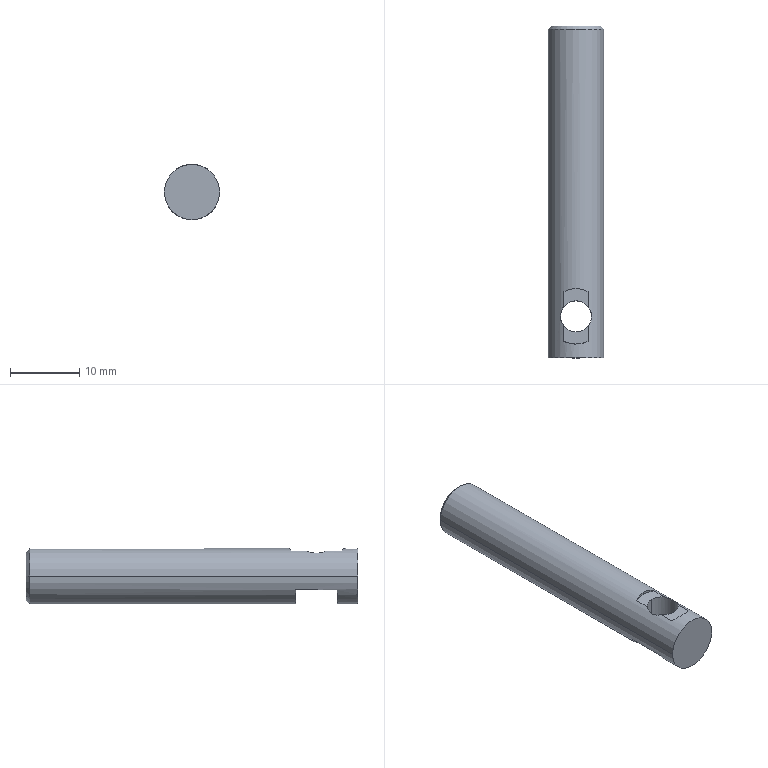Component | SolidWorks | 002MaterialPickingModuleA-1_004SidePlugModule-1_J-014-3 | 1 solid | 20 faces | box 8 x 48 x 8 mm | volume 2217 mm3 | cylinder 9 | plane 7 | cone 4 | commonest cylinder face diameters 8 x5 4.5 x2 2.5 x2 | material 45
build123d program:
from build123d import *

# Parameters (mm, degrees)
SKETCH1_R             = 4
BOSS_EXTRUDE1_DEPTH   = 48
M3_TAPPED_HOLE1_D     = 2.5
M3_TAPPED_HOLE1_DEPTH = 7.5
M3_TAPPED_HOLE1_TIP   = 0.7511
CHAMFER1_SIZE         = 0.5
SKETCH6_W             = 15
SKETCH6_H             = 6
CUT_EXTRUDE1_DEPTH    = 2


with BuildPart() as part:
    # Sketch1 → Boss-Extrude1 (new body)
    with BuildSketch(Plane.XY):
        Circle(SKETCH1_R)
    extrude(amount=BOSS_EXTRUDE1_DEPTH)

    # M3 Tapped Hole1
    with Locations(Plane(origin=(0, 0, 0), x_dir=(-1, 0, 0), z_dir=(0, 0, -1))):
        with Locations((0, 0)):
            Hole(M3_TAPPED_HOLE1_D / 2, depth=M3_TAPPED_HOLE1_DEPTH)
            with Locations((0, 0, -(M3_TAPPED_HOLE1_DEPTH + M3_TAPPED_HOLE1_TIP / 2))):  # 118° drill point
                Cone(0, M3_TAPPED_HOLE1_D / 2, M3_TAPPED_HOLE1_TIP, mode=Mode.SUBTRACT)

    # Chamfer1
    chamfer1_edges = [part.edges().sort_by_distance(p)[0] for p in [
        (-4, 0, 0),
    ]]
    chamfer(chamfer1_edges, length=CHAMFER1_SIZE)

    # Sketch6 → Cut-Extrude1 (cut)
    with BuildSketch(Plane(origin=(0, 4, 0), x_dir=(1, 0, 0), z_dir=(0, 1, 0))):
        with Locations((0, -42)):
            Rectangle(SKETCH6_W, SKETCH6_H)
    extrude(amount=-CUT_EXTRUDE1_DEPTH, mode=Mode.SUBTRACT)

    # Sketch8 → M4 Hex Socket Head Cap Screw CBORE1 (revolve, cut)
    with BuildSketch(Plane(origin=(0, -8, 42), x_dir=(0, 0, -1), z_dir=(1, 0, 0))):
        Polygon((0, 0), (0, 12), (2.25, 12), (2.25, 4.4), (4, 4.4), (4, 0.025), (4.025, 0), align=None)
    revolve(axis=Axis((0, -14.35, 42), (0, 1, 0)), mode=Mode.SUBTRACT)


solid = part.part

# Placed as in the assembly
solid = solid.moved(Location((95.325, 338.019, 464.731), (90, 0, -180)))
STEP:
#1=CARTESIAN_POINT('',(3.753,11.743,18.218));
#2=VERTEX_POINT('',#1);
#3=CARTESIAN_POINT('',(3.753,11.566,18.218));
#4=VERTEX_POINT('',#3);
#5=CARTESIAN_POINT('',(3.753,11.654,18.218));
#6=DIRECTION('',(0.,-0.,-1.));
#7=DIRECTION('',(0.,-1.,0.));
#8=AXIS2_PLACEMENT_3D('',#5,#6,#7);
#9=CIRCLE('',#8,0.08858);
#10=EDGE_CURVE('',#2,#4,#9,.T.);
#11=ORIENTED_EDGE('',*,*,#10,.T.);
#12=CARTESIAN_POINT('',(3.753,11.566,18.438));
#13=VERTEX_POINT('',#12);
#14=CARTESIAN_POINT('',(3.753,11.566,18.611));
#15=DIRECTION('',(-0.,0.,1.));
#16=VECTOR('',#15,39.37);
#17=LINE('',#14,#16);
#18=EDGE_CURVE('',#4,#13,#17,.T.);
#19=ORIENTED_EDGE('',*,*,#18,.T.);
#20=CARTESIAN_POINT('',(3.822,11.598,18.438));
#21=VERTEX_POINT('',#20);
#22=CARTESIAN_POINT('',(3.753,11.654,18.438));
#23=DIRECTION('',(-0.,0.,1.));
#24=DIRECTION('',(0.,1.,0.));
#25=AXIS2_PLACEMENT_3D('',#22,#23,#24);
#26=CIRCLE('',#25,0.08858);
#27=EDGE_CURVE('',#13,#21,#26,.T.);
#28=ORIENTED_EDGE('',*,*,#27,.T.);
#29=CARTESIAN_POINT('',(3.822,11.71,18.438));
#30=VERTEX_POINT('',#29);
#31=CARTESIAN_POINT('',(3.822,11.71,18.438));
#32=CARTESIAN_POINT('',(3.828,11.703,18.435));
#33=CARTESIAN_POINT('',(3.833,11.694,18.432));
#34=CARTESIAN_POINT('',(3.838,11.68,18.429));
#35=CARTESIAN_POINT('',(3.839,11.675,18.428));
#36=CARTESIAN_POINT('',(3.841,11.665,18.427));
#37=CARTESIAN_POINT('',(3.842,11.66,18.427));
#38=CARTESIAN_POINT('',(3.842,11.649,18.427));
#39=CARTESIAN_POINT('',(3.841,11.644,18.427));
#40=CARTESIAN_POINT('',(3.839,11.634,18.428));
#41=CARTESIAN_POINT('',(3.838,11.629,18.429));
#42=CARTESIAN_POINT('',(3.833,11.615,18.432));
#43=CARTESIAN_POINT('',(3.828,11.606,18.435));
#44=CARTESIAN_POINT('',(3.822,11.598,18.438));
#45=B_SPLINE_CURVE_WITH_KNOTS('',3,(#31,#32,#33,#34,#35,#36,#37,#38,#39,#40,#41,#42,#43,#44),.UNSPECIFIED.,.F.,.F.,(4,2,2,2,2,2,4),(0.,0.0007826,0.001174,0.001565,0.001957,0.002348,0.00313),.UNSPECIFIED.);
#46=EDGE_CURVE('',#30,#21,#45,.T.);
#47=ORIENTED_EDGE('',*,*,#46,.F.);
#48=CARTESIAN_POINT('',(3.753,11.743,18.438));
#49=VERTEX_POINT('',#48);
#50=CARTESIAN_POINT('',(3.753,11.654,18.438));
#51=DIRECTION('',(-0.,0.,1.));
#52=DIRECTION('',(0.,1.,0.));
#53=AXIS2_PLACEMENT_3D('',#50,#51,#52);
#54=CIRCLE('',#53,0.08858);
#55=EDGE_CURVE('',#30,#49,#54,.T.);
#56=ORIENTED_EDGE('',*,*,#55,.T.);
#57=CARTESIAN_POINT('',(3.753,11.743,18.611));
#58=DIRECTION('',(-0.,0.,1.));
#59=VECTOR('',#58,39.37);
#60=LINE('',#57,#59);
#61=EDGE_CURVE('',#2,#49,#60,.T.);
#62=ORIENTED_EDGE('',*,*,#61,.F.);
#63=EDGE_LOOP('',(#11,#19,#28,#47,#56,#62));
#64=FACE_OUTER_BOUND('',#63,.T.);
#65=CARTESIAN_POINT('',(3.753,11.654,18.611));
#66=DIRECTION('',(-0.,0.,1.));
#67=DIRECTION('',(0.,1.,0.));
#68=AXIS2_PLACEMENT_3D('',#65,#66,#67);
#69=CYLINDRICAL_SURFACE('',#68,0.08858);
#70=ADVANCED_FACE('',(#64),#69,.F.);
#71=CARTESIAN_POINT('',(3.753,11.812,18.438));
#72=VERTEX_POINT('',#71);
#73=CARTESIAN_POINT('',(3.684,11.796,18.438));
#74=VERTEX_POINT('',#73);
#75=CARTESIAN_POINT('',(3.753,11.654,18.438));
#76=DIRECTION('',(-0.,0.,1.));
#77=DIRECTION('',(0.,1.,0.));
#78=AXIS2_PLACEMENT_3D('',#75,#76,#77);
#79=CIRCLE('',#78,0.1575);
#80=EDGE_CURVE('',#72,#74,#79,.T.);
#81=ORIENTED_EDGE('',*,*,#80,.F.);
#82=CARTESIAN_POINT('',(3.753,11.812,18.454));
#83=VERTEX_POINT('',#82);
#84=CARTESIAN_POINT('',(3.753,11.812,18.611));
#85=DIRECTION('',(-0.,0.,1.));
#86=VECTOR('',#85,39.37);
#87=LINE('',#84,#86);
#88=EDGE_CURVE('',#72,#83,#87,.T.);
#89=ORIENTED_EDGE('',*,*,#88,.T.);
#90=CARTESIAN_POINT('',(3.684,11.796,18.438));
#91=CARTESIAN_POINT('',(3.706,11.806,18.449));
#92=CARTESIAN_POINT('',(3.729,11.812,18.454));
#93=CARTESIAN_POINT('',(3.753,11.812,18.454));
#94=(BOUNDED_CURVE()B_SPLINE_CURVE(3,(#90,#91,#92,#93),.UNSPECIFIED.,.F.,.F.)B_SPLINE_CURVE_WITH_KNOTS((4,4),(5.832,6.283),.UNSPECIFIED.)CURVE()GEOMETRIC_REPRESENTATION_ITEM()RATIONAL_B_SPLINE_CURVE((1.,0.9831,0.9831,1.))REPRESENTATION_ITEM(''));
#95=EDGE_CURVE('',#74,#83,#94,.T.);
#96=ORIENTED_EDGE('',*,*,#95,.F.);
#97=EDGE_LOOP('',(#81,#89,#96));
#98=FACE_OUTER_BOUND('',#97,.T.);
#99=CARTESIAN_POINT('',(3.753,11.654,18.611));
#100=DIRECTION('',(-0.,0.,1.));
#101=DIRECTION('',(0.,1.,0.));
#102=AXIS2_PLACEMENT_3D('',#99,#100,#101);
#103=CYLINDRICAL_SURFACE('',#102,0.1575);
#104=ADVANCED_FACE('',(#98),#103,.F.);
#105=CARTESIAN_POINT('',(3.891,13.308,18.296));
#106=VERTEX_POINT('',#105);
#107=CARTESIAN_POINT('',(3.615,13.308,18.296));
#108=VERTEX_POINT('',#107);
#109=CARTESIAN_POINT('',(3.753,13.308,18.296));
#110=DIRECTION('',(-0.,1.,-0.));
#111=DIRECTION('',(-1.,0.,0.));
#112=AXIS2_PLACEMENT_3D('',#109,#110,#111);
#113=CIRCLE('',#112,0.1378);
#114=EDGE_CURVE('',#106,#108,#113,.T.);
#115=ORIENTED_EDGE('',*,*,#114,.F.);
#116=CARTESIAN_POINT('',(3.91,13.288,18.296));
#117=VERTEX_POINT('',#116);
#118=CARTESIAN_POINT('',(3.91,13.288,18.296));
#119=DIRECTION('',(0.7071,-0.7071,-0.));
#120=VECTOR('',#119,39.37);
#121=LINE('',#118,#120);
#122=EDGE_CURVE('',#106,#117,#121,.T.);
#123=ORIENTED_EDGE('',*,*,#122,.T.);
#124=CARTESIAN_POINT('',(3.595,13.288,18.296));
#125=VERTEX_POINT('',#124);
#126=CARTESIAN_POINT('',(3.753,13.288,18.296));
#127=DIRECTION('',(0.,-1.,0.));
#128=DIRECTION('',(-1.,0.,0.));
#129=AXIS2_PLACEMENT_3D('',#126,#127,#128);
#130=CIRCLE('',#129,0.1575);
#131=EDGE_CURVE('',#125,#117,#130,.T.);
#132=ORIENTED_EDGE('',*,*,#131,.F.);
#133=CARTESIAN_POINT('',(3.595,13.288,18.296));
#134=DIRECTION('',(-0.7071,-0.7071,0.));
#135=VECTOR('',#134,39.37);
#136=LINE('',#133,#135);
#137=EDGE_CURVE('',#108,#125,#136,.T.);
#138=ORIENTED_EDGE('',*,*,#137,.F.);
#139=EDGE_LOOP('',(#115,#123,#132,#138));
#140=FACE_OUTER_BOUND('',#139,.T.);
#141=CARTESIAN_POINT('',(3.753,13.288,18.296));
#142=DIRECTION('',(0.,-1.,0.));
#143=DIRECTION('',(-1.,0.,0.));
#144=AXIS2_PLACEMENT_3D('',#141,#142,#143);
#145=CONICAL_SURFACE('',#144,0.1575,0.7854);
#146=ADVANCED_FACE('',(#140),#145,.T.);
#147=CARTESIAN_POINT('',(3.704,13.013,18.296));
#148=VERTEX_POINT('',#147);
#149=CARTESIAN_POINT('',(3.802,13.013,18.296));
#150=VERTEX_POINT('',#149);
#151=CARTESIAN_POINT('',(3.753,13.013,18.296));
#152=DIRECTION('',(-0.,1.,-0.));
#153=DIRECTION('',(1.,0.,0.));
#154=AXIS2_PLACEMENT_3D('',#151,#152,#153);
#155=CIRCLE('',#154,0.04921);
#156=EDGE_CURVE('',#148,#150,#155,.T.);
#157=ORIENTED_EDGE('',*,*,#156,.F.);
#158=CARTESIAN_POINT('',(3.704,13.308,18.296));
#159=VERTEX_POINT('',#158);
#160=CARTESIAN_POINT('',(3.704,13.308,18.296));
#161=DIRECTION('',(-0.,1.,-0.));
#162=VECTOR('',#161,39.37);
#163=LINE('',#160,#162);
#164=EDGE_CURVE('',#148,#159,#163,.T.);
#165=ORIENTED_EDGE('',*,*,#164,.T.);
#166=CARTESIAN_POINT('',(3.802,13.308,18.296));
#167=VERTEX_POINT('',#166);
#168=CARTESIAN_POINT('',(3.753,13.308,18.296));
#169=DIRECTION('',(-0.,1.,-0.));
#170=DIRECTION('',(1.,0.,0.));
#171=AXIS2_PLACEMENT_3D('',#168,#169,#170);
#172=CIRCLE('',#171,0.04921);
#173=EDGE_CURVE('',#159,#167,#172,.T.);
#174=ORIENTED_EDGE('',*,*,#173,.T.);
#175=CARTESIAN_POINT('',(3.802,13.308,18.296));
#176=DIRECTION('',(-0.,1.,-0.));
#177=VECTOR('',#176,39.37);
#178=LINE('',#175,#177);
#179=EDGE_CURVE('',#150,#167,#178,.T.);
#180=ORIENTED_EDGE('',*,*,#179,.F.);
#181=EDGE_LOOP('',(#157,#165,#174,#180));
#182=FACE_OUTER_BOUND('',#181,.T.);
#183=CARTESIAN_POINT('',(3.753,13.308,18.296));
#184=DIRECTION('',(-0.,1.,-0.));
#185=DIRECTION('',(1.,0.,0.));
#186=AXIS2_PLACEMENT_3D('',#183,#184,#185);
#187=CYLINDRICAL_SURFACE('',#186,0.04921);
#188=ADVANCED_FACE('',(#182),#187,.F.);
#189=CARTESIAN_POINT('',(3.753,12.983,18.296));
#190=VERTEX_POINT('',#189);
#191=CARTESIAN_POINT('',(3.802,13.013,18.296));
#192=DIRECTION('',(0.8572,0.515,-0.));
#193=VECTOR('',#192,39.37);
#194=LINE('',#191,#193);
#195=EDGE_CURVE('',#190,#150,#194,.T.);
#196=ORIENTED_EDGE('',*,*,#195,.F.);
#197=CARTESIAN_POINT('',(3.704,13.013,18.296));
#198=DIRECTION('',(-0.8572,0.515,-0.));
#199=VECTOR('',#198,39.37);
#200=LINE('',#197,#199);
#201=EDGE_CURVE('',#190,#148,#200,.T.);
#202=ORIENTED_EDGE('',*,*,#201,.T.);
#203=ORIENTED_EDGE('',*,*,#156,.T.);
#204=EDGE_LOOP('',(#196,#202,#203));
#205=FACE_OUTER_BOUND('',#204,.T.);
#206=CARTESIAN_POINT('',(3.753,13.013,18.296));
#207=DIRECTION('',(-0.,1.,-0.));
#208=DIRECTION('',(1.,0.,0.));
#209=AXIS2_PLACEMENT_3D('',#206,#207,#208);
#210=CONICAL_SURFACE('',#209,0.04921,1.03);
#211=ADVANCED_FACE('',(#205),#210,.F.);
#212=CARTESIAN_POINT('',(3.889,11.772,18.218));
#213=VERTEX_POINT('',#212);
#214=CARTESIAN_POINT('',(3.889,11.536,18.218));
#215=VERTEX_POINT('',#214);
#216=CARTESIAN_POINT('',(3.889,11.418,18.218));
#217=DIRECTION('',(0.,-1.,0.));
#218=VECTOR('',#217,39.37);
#219=LINE('',#216,#218);
#220=EDGE_CURVE('',#213,#215,#219,.T.);
#221=ORIENTED_EDGE('',*,*,#220,.F.);
#222=CARTESIAN_POINT('',(3.617,11.772,18.218));
#223=VERTEX_POINT('',#222);
#224=CARTESIAN_POINT('',(3.753,11.772,18.296));
#225=DIRECTION('',(-0.,1.,-0.));
#226=DIRECTION('',(1.,0.,0.));
#227=AXIS2_PLACEMENT_3D('',#224,#225,#226);
#228=CIRCLE('',#227,0.1575);
#229=EDGE_CURVE('',#213,#223,#228,.T.);
#230=ORIENTED_EDGE('',*,*,#229,.T.);
#231=CARTESIAN_POINT('',(3.617,11.536,18.218));
#232=VERTEX_POINT('',#231);
#233=CARTESIAN_POINT('',(3.617,11.418,18.218));
#234=DIRECTION('',(-0.,1.,-0.));
#235=VECTOR('',#234,39.37);
#236=LINE('',#233,#235);
#237=EDGE_CURVE('',#232,#223,#236,.T.);
#238=ORIENTED_EDGE('',*,*,#237,.F.);
#239=CARTESIAN_POINT('',(3.753,11.536,18.296));
#240=DIRECTION('',(0.,-1.,0.));
#241=DIRECTION('',(-1.,0.,0.));
#242=AXIS2_PLACEMENT_3D('',#239,#240,#241);
#243=CIRCLE('',#242,0.1575);
#244=EDGE_CURVE('',#232,#215,#243,.T.);
#245=ORIENTED_EDGE('',*,*,#244,.T.);
#246=EDGE_LOOP('',(#221,#230,#238,#245));
#247=FACE_BOUND('',#246,.T.);
#248=CARTESIAN_POINT('',(3.595,11.418,18.296));
#249=VERTEX_POINT('',#248);
#250=CARTESIAN_POINT('',(3.91,11.418,18.296));
#251=VERTEX_POINT('',#250);
#252=CARTESIAN_POINT('',(3.753,11.418,18.296));
#253=DIRECTION('',(0.,-1.,0.));
#254=DIRECTION('',(-1.,0.,0.));
#255=AXIS2_PLACEMENT_3D('',#252,#253,#254);
#256=CIRCLE('',#255,0.1575);
#257=EDGE_CURVE('',#249,#251,#256,.T.);
#258=ORIENTED_EDGE('',*,*,#257,.F.);
#259=CARTESIAN_POINT('',(3.595,11.418,18.296));
#260=DIRECTION('',(-0.,1.,-0.));
#261=VECTOR('',#260,39.37);
#262=LINE('',#259,#261);
#263=EDGE_CURVE('',#249,#125,#262,.T.);
#264=ORIENTED_EDGE('',*,*,#263,.T.);
#265=ORIENTED_EDGE('',*,*,#131,.T.);
#266=CARTESIAN_POINT('',(3.91,11.418,18.296));
#267=DIRECTION('',(-0.,1.,-0.));
#268=VECTOR('',#267,39.37);
#269=LINE('',#266,#268);
#270=EDGE_CURVE('',#251,#117,#269,.T.);
#271=ORIENTED_EDGE('',*,*,#270,.F.);
#272=EDGE_LOOP('',(#258,#264,#265,#271));
#273=FACE_OUTER_BOUND('',#272,.T.);
#274=CARTESIAN_POINT('',(3.753,11.418,18.296));
#275=DIRECTION('',(-0.,1.,-0.));
#276=DIRECTION('',(1.,0.,0.));
#277=AXIS2_PLACEMENT_3D('',#274,#275,#276);
#278=CYLINDRICAL_SURFACE('',#277,0.1575);
#279=ADVANCED_FACE('',(#247,#273),#278,.T.);
#280=ORIENTED_EDGE('',*,*,#263,.F.);
#281=CARTESIAN_POINT('',(3.753,11.418,18.296));
#282=DIRECTION('',(0.,-1.,0.));
#283=DIRECTION('',(-1.,0.,0.));
#284=AXIS2_PLACEMENT_3D('',#281,#282,#283);
#285=CIRCLE('',#284,0.1575);
#286=EDGE_CURVE('',#251,#249,#285,.T.);
#287=ORIENTED_EDGE('',*,*,#286,.F.);
#288=ORIENTED_EDGE('',*,*,#270,.T.);
#289=CARTESIAN_POINT('',(3.753,13.288,18.296));
#290=DIRECTION('',(0.,-1.,0.));
#291=DIRECTION('',(-1.,0.,0.));
#292=AXIS2_PLACEMENT_3D('',#289,#290,#291);
#293=CIRCLE('',#292,0.1575);
#294=EDGE_CURVE('',#117,#125,#293,.T.);
#295=ORIENTED_EDGE('',*,*,#294,.T.);
#296=EDGE_LOOP('',(#280,#287,#288,#295));
#297=FACE_OUTER_BOUND('',#296,.T.);
#298=CARTESIAN_POINT('',(3.684,11.513,18.438));
#299=VERTEX_POINT('',#298);
#300=CARTESIAN_POINT('',(3.684,11.598,18.438));
#301=VERTEX_POINT('',#300);
#302=CARTESIAN_POINT('',(3.684,11.418,18.438));
#303=DIRECTION('',(-0.,1.,-0.));
#304=VECTOR('',#303,39.37);
#305=LINE('',#302,#304);
#306=EDGE_CURVE('',#299,#301,#305,.T.);
#307=ORIENTED_EDGE('',*,*,#306,.T.);
#308=CARTESIAN_POINT('',(3.684,11.71,18.438));
#309=VERTEX_POINT('',#308);
#310=CARTESIAN_POINT('',(3.684,11.598,18.438));
#311=CARTESIAN_POINT('',(3.678,11.606,18.435));
#312=CARTESIAN_POINT('',(3.673,11.615,18.432));
#313=CARTESIAN_POINT('',(3.668,11.629,18.429));
#314=CARTESIAN_POINT('',(3.667,11.634,18.428));
#315=CARTESIAN_POINT('',(3.665,11.644,18.427));
#316=CARTESIAN_POINT('',(3.664,11.649,18.427));
#317=CARTESIAN_POINT('',(3.664,11.659,18.427));
#318=CARTESIAN_POINT('',(3.665,11.664,18.427));
#319=CARTESIAN_POINT('',(3.667,11.675,18.428));
#320=CARTESIAN_POINT('',(3.668,11.68,18.429));
#321=CARTESIAN_POINT('',(3.673,11.694,18.432));
#322=CARTESIAN_POINT('',(3.678,11.703,18.435));
#323=CARTESIAN_POINT('',(3.684,11.71,18.438));
#324=B_SPLINE_CURVE_WITH_KNOTS('',3,(#310,#311,#312,#313,#314,#315,#316,#317,#318,#319,#320,#321,#322,#323),.UNSPECIFIED.,.F.,.F.,(4,2,2,2,2,2,4),(0.,0.0007826,0.001174,0.001565,0.001957,0.002348,0.00313),.UNSPECIFIED.);
#325=EDGE_CURVE('',#301,#309,#324,.T.);
#326=ORIENTED_EDGE('',*,*,#325,.T.);
#327=CARTESIAN_POINT('',(3.684,11.418,18.438));
#328=DIRECTION('',(-0.,1.,-0.));
#329=VECTOR('',#328,39.37);
#330=LINE('',#327,#329);
#331=EDGE_CURVE('',#309,#74,#330,.T.);
#332=ORIENTED_EDGE('',*,*,#331,.T.);
#333=ORIENTED_EDGE('',*,*,#95,.T.);
#334=CARTESIAN_POINT('',(3.822,11.796,18.438));
#335=VERTEX_POINT('',#334);
#336=CARTESIAN_POINT('',(3.753,11.812,18.454));
#337=CARTESIAN_POINT('',(3.777,11.812,18.454));
#338=CARTESIAN_POINT('',(3.8,11.806,18.449));
#339=CARTESIAN_POINT('',(3.822,11.796,18.438));
#340=(BOUNDED_CURVE()B_SPLINE_CURVE(3,(#336,#337,#338,#339),.UNSPECIFIED.,.F.,.F.)B_SPLINE_CURVE_WITH_KNOTS((4,4),(0.,0.451),.UNSPECIFIED.)CURVE()GEOMETRIC_REPRESENTATION_ITEM()RATIONAL_B_SPLINE_CURVE((1.,0.9831,0.9831,1.))REPRESENTATION_ITEM(''));
#341=EDGE_CURVE('',#83,#335,#340,.T.);
#342=ORIENTED_EDGE('',*,*,#341,.T.);
#343=CARTESIAN_POINT('',(3.822,11.418,18.438));
#344=DIRECTION('',(0.,-1.,0.));
#345=VECTOR('',#344,39.37);
#346=LINE('',#343,#345);
#347=EDGE_CURVE('',#335,#30,#346,.T.);
#348=ORIENTED_EDGE('',*,*,#347,.T.);
#349=ORIENTED_EDGE('',*,*,#46,.T.);
#350=CARTESIAN_POINT('',(3.822,11.513,18.438));
#351=VERTEX_POINT('',#350);
#352=CARTESIAN_POINT('',(3.822,11.418,18.438));
#353=DIRECTION('',(0.,-1.,0.));
#354=VECTOR('',#353,39.37);
#355=LINE('',#352,#354);
#356=EDGE_CURVE('',#21,#351,#355,.T.);
#357=ORIENTED_EDGE('',*,*,#356,.T.);
#358=CARTESIAN_POINT('',(3.822,11.513,18.438));
#359=CARTESIAN_POINT('',(3.777,11.491,18.46));
#360=CARTESIAN_POINT('',(3.728,11.491,18.46));
#361=CARTESIAN_POINT('',(3.684,11.513,18.438));
#362=(BOUNDED_CURVE()B_SPLINE_CURVE(3,(#358,#359,#360,#361),.UNSPECIFIED.,.F.,.F.)B_SPLINE_CURVE_WITH_KNOTS((4,4),(2.691,3.593),.UNSPECIFIED.)CURVE()GEOMETRIC_REPRESENTATION_ITEM()RATIONAL_B_SPLINE_CURVE((1.,0.9333,0.9333,1.))REPRESENTATION_ITEM(''));
#363=EDGE_CURVE('',#351,#299,#362,.T.);
#364=ORIENTED_EDGE('',*,*,#363,.T.);
#365=EDGE_LOOP('',(#307,#326,#332,#333,#342,#348,#349,#357,#364));
#366=FACE_BOUND('',#365,.T.);
#367=CARTESIAN_POINT('',(3.753,11.418,18.296));
#368=DIRECTION('',(-0.,1.,-0.));
#369=DIRECTION('',(1.,0.,0.));
#370=AXIS2_PLACEMENT_3D('',#367,#368,#369);
#371=CYLINDRICAL_SURFACE('',#370,0.1575);
#372=ADVANCED_FACE('',(#297,#366),#371,.T.);
#373=ORIENTED_EDGE('',*,*,#286,.T.);
#374=ORIENTED_EDGE('',*,*,#257,.T.);
#375=EDGE_LOOP('',(#373,#374));
#376=FACE_OUTER_BOUND('',#375,.T.);
#377=CARTESIAN_POINT('',(3.753,11.418,18.296));
#378=DIRECTION('',(-0.,-1.,0.));
#379=DIRECTION('',(-1.,-0.,-0.));
#380=AXIS2_PLACEMENT_3D('',#377,#378,#379);
#381=PLANE('',#380);
#382=ADVANCED_FACE('',(#376),#381,.T.);
#383=CARTESIAN_POINT('',(3.753,13.308,18.296));
#384=DIRECTION('',(-0.,1.,-0.));
#385=DIRECTION('',(-1.,0.,0.));
#386=AXIS2_PLACEMENT_3D('',#383,#384,#385);
#387=CIRCLE('',#386,0.1378);
#388=EDGE_CURVE('',#108,#106,#387,.T.);
#389=ORIENTED_EDGE('',*,*,#388,.T.);
#390=ORIENTED_EDGE('',*,*,#114,.T.);
#391=EDGE_LOOP('',(#389,#390));
#392=FACE_OUTER_BOUND('',#391,.T.);
#393=CARTESIAN_POINT('',(3.753,13.308,18.296));
#394=DIRECTION('',(-0.,1.,-0.));
#395=DIRECTION('',(1.,0.,0.));
#396=AXIS2_PLACEMENT_3D('',#393,#394,#395);
#397=CIRCLE('',#396,0.04921);
#398=EDGE_CURVE('',#167,#159,#397,.T.);
#399=ORIENTED_EDGE('',*,*,#398,.F.);
#400=ORIENTED_EDGE('',*,*,#173,.F.);
#401=EDGE_LOOP('',(#399,#400));
#402=FACE_BOUND('',#401,.T.);
#403=CARTESIAN_POINT('',(3.753,13.308,18.296));
#404=DIRECTION('',(-0.,-1.,0.));
#405=DIRECTION('',(-1.,-0.,-0.));
#406=AXIS2_PLACEMENT_3D('',#403,#404,#405);
#407=PLANE('',#406);
#408=ADVANCED_FACE('',(#392,#402),#407,.F.);
#409=ORIENTED_EDGE('',*,*,#201,.F.);
#410=ORIENTED_EDGE('',*,*,#195,.T.);
#411=CARTESIAN_POINT('',(3.753,13.013,18.296));
#412=DIRECTION('',(-0.,1.,-0.));
#413=DIRECTION('',(1.,0.,0.));
#414=AXIS2_PLACEMENT_3D('',#411,#412,#413);
#415=CIRCLE('',#414,0.04921);
#416=EDGE_CURVE('',#150,#148,#415,.T.);
#417=ORIENTED_EDGE('',*,*,#416,.T.);
#418=EDGE_LOOP('',(#409,#410,#417));
#419=FACE_OUTER_BOUND('',#418,.T.);
#420=CARTESIAN_POINT('',(3.753,13.013,18.296));
#421=DIRECTION('',(-0.,1.,-0.));
#422=DIRECTION('',(1.,0.,0.));
#423=AXIS2_PLACEMENT_3D('',#420,#421,#422);
#424=CONICAL_SURFACE('',#423,0.04921,1.03);
#425=ADVANCED_FACE('',(#419),#424,.F.);
#426=ORIENTED_EDGE('',*,*,#164,.F.);
#427=ORIENTED_EDGE('',*,*,#416,.F.);
#428=ORIENTED_EDGE('',*,*,#179,.T.);
#429=ORIENTED_EDGE('',*,*,#398,.T.);
#430=EDGE_LOOP('',(#426,#427,#428,#429));
#431=FACE_OUTER_BOUND('',#430,.T.);
#432=CARTESIAN_POINT('',(3.753,13.308,18.296));
#433=DIRECTION('',(-0.,1.,-0.));
#434=DIRECTION('',(1.,0.,0.));
#435=AXIS2_PLACEMENT_3D('',#432,#433,#434);
#436=CYLINDRICAL_SURFACE('',#435,0.04921);
#437=ADVANCED_FACE('',(#431),#436,.F.);
#438=ORIENTED_EDGE('',*,*,#122,.F.);
#439=ORIENTED_EDGE('',*,*,#388,.F.);
#440=ORIENTED_EDGE('',*,*,#137,.T.);
#441=ORIENTED_EDGE('',*,*,#294,.F.);
#442=EDGE_LOOP('',(#438,#439,#440,#441));
#443=FACE_OUTER_BOUND('',#442,.T.);
#444=CARTESIAN_POINT('',(3.753,13.288,18.296));
#445=DIRECTION('',(0.,-1.,0.));
#446=DIRECTION('',(-1.,0.,0.));
#447=AXIS2_PLACEMENT_3D('',#444,#445,#446);
#448=CONICAL_SURFACE('',#447,0.1575,0.7854);
#449=ADVANCED_FACE('',(#443),#448,.T.);
#450=CARTESIAN_POINT('',(3.458,11.772,18.218));
#451=DIRECTION('',(1.,0.,0.));
#452=VECTOR('',#451,39.37);
#453=LINE('',#450,#452);
#454=EDGE_CURVE('',#223,#213,#453,.T.);
#455=ORIENTED_EDGE('',*,*,#454,.F.);
#456=ORIENTED_EDGE('',*,*,#229,.F.);
#457=EDGE_LOOP('',(#455,#456));
#458=FACE_OUTER_BOUND('',#457,.T.);
#459=CARTESIAN_POINT('',(3.458,11.772,18.218));
#460=DIRECTION('',(0.,1.,-0.));
#461=DIRECTION('',(1.,0.,0.));
#462=AXIS2_PLACEMENT_3D('',#459,#460,#461);
#463=PLANE('',#462);
#464=ADVANCED_FACE('',(#458),#463,.F.);
#465=CARTESIAN_POINT('',(3.458,11.536,18.218));
#466=DIRECTION('',(-1.,-0.,-0.));
#467=VECTOR('',#466,39.37);
#468=LINE('',#465,#467);
#469=EDGE_CURVE('',#215,#232,#468,.T.);
#470=ORIENTED_EDGE('',*,*,#469,.F.);
#471=ORIENTED_EDGE('',*,*,#244,.F.);
#472=EDGE_LOOP('',(#470,#471));
#473=FACE_OUTER_BOUND('',#472,.T.);
#474=CARTESIAN_POINT('',(3.458,11.536,18.218));
#475=DIRECTION('',(-0.,-1.,0.));
#476=DIRECTION('',(-1.,-0.,-0.));
#477=AXIS2_PLACEMENT_3D('',#474,#475,#476);
#478=PLANE('',#477);
#479=ADVANCED_FACE('',(#473),#478,.F.);
#480=ORIENTED_EDGE('',*,*,#10,.F.);
#481=CARTESIAN_POINT('',(3.753,11.654,18.218));
#482=DIRECTION('',(0.,-0.,-1.));
#483=DIRECTION('',(0.,-1.,0.));
#484=AXIS2_PLACEMENT_3D('',#481,#482,#483);
#485=CIRCLE('',#484,0.08858);
#486=EDGE_CURVE('',#4,#2,#485,.T.);
#487=ORIENTED_EDGE('',*,*,#486,.F.);
#488=EDGE_LOOP('',(#480,#487));
#489=FACE_BOUND('',#488,.T.);
#490=ORIENTED_EDGE('',*,*,#237,.T.);
#491=ORIENTED_EDGE('',*,*,#454,.T.);
#492=ORIENTED_EDGE('',*,*,#220,.T.);
#493=ORIENTED_EDGE('',*,*,#469,.T.);
#494=EDGE_LOOP('',(#490,#491,#492,#493));
#495=FACE_OUTER_BOUND('',#494,.T.);
#496=CARTESIAN_POINT('',(3.753,13.308,18.218));
#497=DIRECTION('',(0.,-0.,-1.));
#498=DIRECTION('',(0.,-1.,0.));
#499=AXIS2_PLACEMENT_3D('',#496,#497,#498);
#500=PLANE('',#499);
#501=ADVANCED_FACE('',(#489,#495),#500,.T.);
#502=CARTESIAN_POINT('',(3.753,11.654,18.438));
#503=DIRECTION('',(-0.,0.,1.));
#504=DIRECTION('',(0.,1.,0.));
#505=AXIS2_PLACEMENT_3D('',#502,#503,#504);
#506=CIRCLE('',#505,0.1575);
#507=EDGE_CURVE('',#299,#351,#506,.T.);
#508=ORIENTED_EDGE('',*,*,#507,.T.);
#509=ORIENTED_EDGE('',*,*,#356,.F.);
#510=ORIENTED_EDGE('',*,*,#27,.F.);
#511=CARTESIAN_POINT('',(3.753,11.654,18.438));
#512=DIRECTION('',(-0.,0.,1.));
#513=DIRECTION('',(0.,1.,0.));
#514=AXIS2_PLACEMENT_3D('',#511,#512,#513);
#515=CIRCLE('',#514,0.08858);
#516=EDGE_CURVE('',#301,#13,#515,.T.);
#517=ORIENTED_EDGE('',*,*,#516,.F.);
#518=ORIENTED_EDGE('',*,*,#306,.F.);
#519=EDGE_LOOP('',(#508,#509,#510,#517,#518));
#520=FACE_OUTER_BOUND('',#519,.T.);
#521=CARTESIAN_POINT('',(3.595,11.654,18.438));
#522=DIRECTION('',(0.,-0.,-1.));
#523=DIRECTION('',(0.,-1.,0.));
#524=AXIS2_PLACEMENT_3D('',#521,#522,#523);
#525=PLANE('',#524);
#526=ADVANCED_FACE('',(#520),#525,.F.);
#527=ORIENTED_EDGE('',*,*,#55,.F.);
#528=ORIENTED_EDGE('',*,*,#347,.F.);
#529=CARTESIAN_POINT('',(3.753,11.654,18.438));
#530=DIRECTION('',(-0.,0.,1.));
#531=DIRECTION('',(0.,1.,0.));
#532=AXIS2_PLACEMENT_3D('',#529,#530,#531);
#533=CIRCLE('',#532,0.1575);
#534=EDGE_CURVE('',#335,#72,#533,.T.);
#535=ORIENTED_EDGE('',*,*,#534,.T.);
#536=ORIENTED_EDGE('',*,*,#80,.T.);
#537=ORIENTED_EDGE('',*,*,#331,.F.);
#538=CARTESIAN_POINT('',(3.753,11.654,18.438));
#539=DIRECTION('',(-0.,0.,1.));
#540=DIRECTION('',(0.,1.,0.));
#541=AXIS2_PLACEMENT_3D('',#538,#539,#540);
#542=CIRCLE('',#541,0.08858);
#543=EDGE_CURVE('',#49,#309,#542,.T.);
#544=ORIENTED_EDGE('',*,*,#543,.F.);
#545=EDGE_LOOP('',(#527,#528,#535,#536,#537,#544));
#546=FACE_OUTER_BOUND('',#545,.T.);
#547=CARTESIAN_POINT('',(3.595,11.654,18.438));
#548=DIRECTION('',(0.,-0.,-1.));
#549=DIRECTION('',(0.,-1.,0.));
#550=AXIS2_PLACEMENT_3D('',#547,#548,#549);
#551=PLANE('',#550);
#552=ADVANCED_FACE('',(#546),#551,.F.);
#553=ORIENTED_EDGE('',*,*,#507,.F.);
#554=ORIENTED_EDGE('',*,*,#363,.F.);
#555=EDGE_LOOP('',(#553,#554));
#556=FACE_OUTER_BOUND('',#555,.T.);
#557=CARTESIAN_POINT('',(3.753,11.654,18.611));
#558=DIRECTION('',(-0.,0.,1.));
#559=DIRECTION('',(0.,1.,0.));
#560=AXIS2_PLACEMENT_3D('',#557,#558,#559);
#561=CYLINDRICAL_SURFACE('',#560,0.1575);
#562=ADVANCED_FACE('',(#556),#561,.F.);
#563=ORIENTED_EDGE('',*,*,#88,.F.);
#564=ORIENTED_EDGE('',*,*,#534,.F.);
#565=ORIENTED_EDGE('',*,*,#341,.F.);
#566=EDGE_LOOP('',(#563,#564,#565));
#567=FACE_OUTER_BOUND('',#566,.T.);
#568=CARTESIAN_POINT('',(3.753,11.654,18.611));
#569=DIRECTION('',(-0.,0.,1.));
#570=DIRECTION('',(0.,1.,0.));
#571=AXIS2_PLACEMENT_3D('',#568,#569,#570);
#572=CYLINDRICAL_SURFACE('',#571,0.1575);
#573=ADVANCED_FACE('',(#567),#572,.F.);
#574=ORIENTED_EDGE('',*,*,#18,.F.);
#575=ORIENTED_EDGE('',*,*,#486,.T.);
#576=ORIENTED_EDGE('',*,*,#61,.T.);
#577=ORIENTED_EDGE('',*,*,#543,.T.);
#578=ORIENTED_EDGE('',*,*,#325,.F.);
#579=ORIENTED_EDGE('',*,*,#516,.T.);
#580=EDGE_LOOP('',(#574,#575,#576,#577,#578,#579));
#581=FACE_OUTER_BOUND('',#580,.T.);
#582=CARTESIAN_POINT('',(3.753,11.654,18.611));
#583=DIRECTION('',(-0.,0.,1.));
#584=DIRECTION('',(0.,1.,0.));
#585=AXIS2_PLACEMENT_3D('',#582,#583,#584);
#586=CYLINDRICAL_SURFACE('',#585,0.08858);
#587=ADVANCED_FACE('',(#581),#586,.F.);
#588=CLOSED_SHELL('',(#70,#104,#146,#188,#211,#279,#372,#382,#408,#425,#437,#449,#464,#479,#501,#526,#552,#562,#573,#587));
#589=MANIFOLD_SOLID_BREP('',#588);
#590=CARTESIAN_POINT('',(0.,0.,0.));
#591=DIRECTION('',(0.,0.,1.));
#592=DIRECTION('',(1.,0.,0.));
#593=AXIS2_PLACEMENT_3D('',#590,#591,#592);
#594=(LENGTH_UNIT()NAMED_UNIT(*)SI_UNIT($,.METRE.));
#595=LENGTH_MEASURE_WITH_UNIT(LENGTH_MEASURE(0.0254),#594);
#596=DIMENSIONAL_EXPONENTS(1.,0.,0.,0.,0.,0.,0.);
#597=(CONVERSION_BASED_UNIT('',#595)LENGTH_UNIT()NAMED_UNIT(#596));
#598=UNCERTAINTY_MEASURE_WITH_UNIT(LENGTH_MEASURE(0.00001),#597,'','');
#599=(NAMED_UNIT(*)PLANE_ANGLE_UNIT()SI_UNIT($,.RADIAN.));
#600=(NAMED_UNIT(*)SI_UNIT($,.STERADIAN.)SOLID_ANGLE_UNIT());
#601=(GEOMETRIC_REPRESENTATION_CONTEXT(3)GLOBAL_UNCERTAINTY_ASSIGNED_CONTEXT((#598))GLOBAL_UNIT_ASSIGNED_CONTEXT((#597,#599,#600))REPRESENTATION_CONTEXT('',''));
#602=ADVANCED_BREP_SHAPE_REPRESENTATION('',(#589,#593),#601);
#603=COLOUR_RGB('',0.7922,0.8196,0.9333);
#604=FILL_AREA_STYLE_COLOUR('',#603);
#605=FILL_AREA_STYLE('',(#604));
#606=SURFACE_STYLE_FILL_AREA(#605);
#607=SURFACE_SIDE_STYLE('',(#606));
#608=SURFACE_STYLE_USAGE(.BOTH.,#607);
#609=PRESENTATION_STYLE_ASSIGNMENT((#608));
#610=STYLED_ITEM('',(#609),#589);
#611=PRESENTATION_LAYER_ASSIGNMENT('','',(#610));
#612=(LENGTH_UNIT()NAMED_UNIT(*)SI_UNIT($,.METRE.));
#613=LENGTH_MEASURE_WITH_UNIT(LENGTH_MEASURE(0.0254),#612);
#614=DIMENSIONAL_EXPONENTS(1.,0.,0.,0.,0.,0.,0.);
#615=(CONVERSION_BASED_UNIT('',#613)LENGTH_UNIT()NAMED_UNIT(#614));
#616=UNCERTAINTY_MEASURE_WITH_UNIT(LENGTH_MEASURE(0.00001),#615,'','');
#617=(NAMED_UNIT(*)PLANE_ANGLE_UNIT()SI_UNIT($,.RADIAN.));
#618=(NAMED_UNIT(*)SI_UNIT($,.STERADIAN.)SOLID_ANGLE_UNIT());
#619=(GEOMETRIC_REPRESENTATION_CONTEXT(3)GLOBAL_UNCERTAINTY_ASSIGNED_CONTEXT((#616))GLOBAL_UNIT_ASSIGNED_CONTEXT((#615,#617,#618))REPRESENTATION_CONTEXT('',''));
#620=MECHANICAL_DESIGN_GEOMETRIC_PRESENTATION_REPRESENTATION('',(#610),#619);